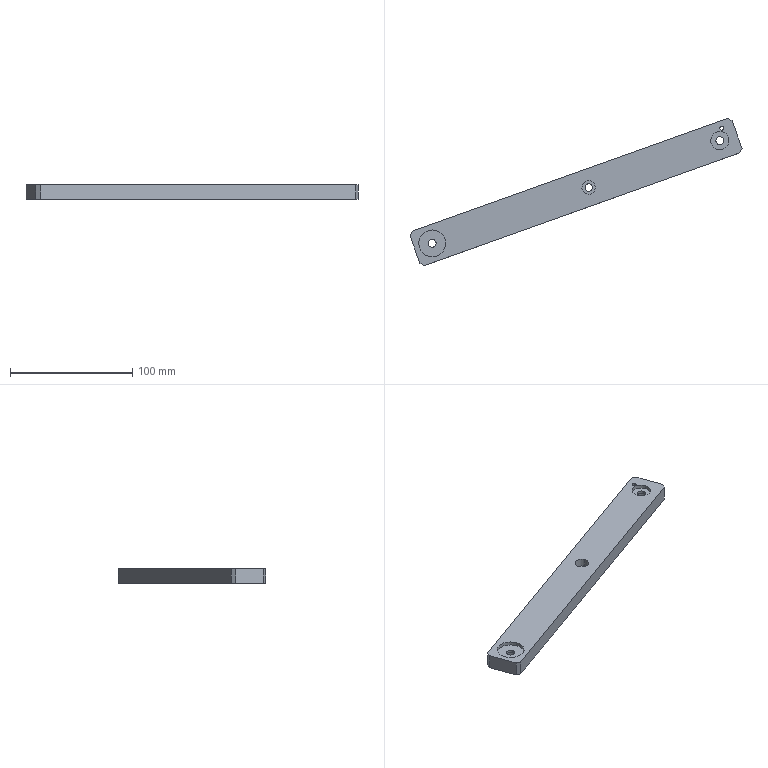Component | SolidWorks | JYTBJ-HeaderBrakeLever-1 | 1 solid | 36 faces | box 271.74 x 120.46 x 12 mm | volume 96229 mm3 | cylinder 20 | plane 16 | commonest cylinder face diameters 11 x6 6.6 x4 3.3 x2 16 x2 22 x2 15 x2 6 x2
build123d program:
from build123d import *

# Parameters (mm, degrees)
SKETCH1_W                                            = 280
SKETCH1_H                                            = 30
BOSS_EXTRUDE1_DEPTH                                  = 12
HOLE_SIZE_ACCORDING_TO_THE_TYPE_OF_HEXAG_D           = 6.6
HOLE_SIZE_ACCORDING_TO_THE_TYPE_OF_HEXAG_CBORE_D     = 11
HOLE_SIZE_ACCORDING_TO_THE_TYPE_OF_HEXAG_CBORE_DEPTH = 6.8
HOLE_SIZE_ACCORDING_TO_THE_TYPE_OF_H_2_D             = 6
HOLE_SIZE_ACCORDING_TO_THE_TYPE_OF_H_2_CBORE_D       = 11
HOLE_SIZE_ACCORDING_TO_THE_TYPE_OF_H_2_CBORE_DEPTH   = 6.8
SKETCH8_R                                            = 7.5
SKETCH8_R_2                                          = 11
CUT_EXTRUDE1_DEPTH                                   = 3
SKETCH9_R                                            = 8
CUT_EXTRUDE2_DEPTH                                   = 2
M4_TAPPED_HOLE1_D                                    = 3.3
CHAMFER1_SIZE                                        = 3


with BuildPart() as part:
    # Sketch1 → Boss-Extrude1 (new body)
    with BuildSketch(Plane.XY):
        Rectangle(SKETCH1_W, SKETCH1_H)
    extrude(amount=BOSS_EXTRUDE1_DEPTH)

    # Hole Size according to the type of hexag (through all)
    with Locations(Plane(origin=(0, 0, 0), x_dir=(-1, 0, 0), z_dir=(0, 0, -1))):
        with Locations((-125, 0), (125, 0)):
            CounterBoreHole(HOLE_SIZE_ACCORDING_TO_THE_TYPE_OF_HEXAG_D / 2, HOLE_SIZE_ACCORDING_TO_THE_TYPE_OF_HEXAG_CBORE_D / 2, HOLE_SIZE_ACCORDING_TO_THE_TYPE_OF_HEXAG_CBORE_DEPTH)

    # Hole Size according to the type of h 2 (through all)
    with Locations(Plane.XY.offset(12)):
        with Locations((-11, 0)):
            CounterBoreHole(HOLE_SIZE_ACCORDING_TO_THE_TYPE_OF_H_2_D / 2, HOLE_SIZE_ACCORDING_TO_THE_TYPE_OF_H_2_CBORE_D / 2, HOLE_SIZE_ACCORDING_TO_THE_TYPE_OF_H_2_CBORE_DEPTH)

    # Sketch8 → Cut-Extrude1 (cut)
    with BuildSketch(Plane.XY.offset(12)):
        with Locations((-125, 0)):
            Circle(SKETCH8_R)
        with Locations((125, 0)):
            Circle(SKETCH8_R_2)
    extrude(amount=-CUT_EXTRUDE1_DEPTH, mode=Mode.SUBTRACT)

    # Sketch9 → Cut-Extrude2 (cut)
    with BuildSketch(Plane(origin=(0, 0, 0), x_dir=(-1, 0, 0), z_dir=(0, 0, -1))):
        with Locations((11, 0)):
            Circle(SKETCH9_R)
    extrude(amount=-CUT_EXTRUDE2_DEPTH, mode=Mode.SUBTRACT)

    # M4 Tapped Hole1 (through all)
    with Locations(Plane(origin=(0, 0, 0), x_dir=(-1, 0, 0), z_dir=(0, 0, -1))):
        with Locations((130, -9)):
            Hole(M4_TAPPED_HOLE1_D / 2)

    # Chamfer1
    chamfer1_edges = [part.edges().sort_by_distance(p)[0] for p in [
        (140, 15, 6),
        (140, -15, 6),
        (-140, -15, 6),
        (-140, 15, 6),
    ]]
    chamfer(chamfer1_edges, length=CHAMFER1_SIZE)


solid = part.part

# Placed as in the assembly
solid = solid.moved(Location((-81.985, 223.08, 9), (0, 0, -160.334)))
STEP:
#1=COLOUR_RGB('',0.7922,0.8196,0.9333);
#2=FILL_AREA_STYLE_COLOUR('',#1);
#3=FILL_AREA_STYLE('',(#2));
#4=SURFACE_STYLE_FILL_AREA(#3);
#5=SURFACE_SIDE_STYLE('',(#4));
#6=SURFACE_STYLE_USAGE(.BOTH.,#5);
#7=PRESENTATION_STYLE_ASSIGNMENT((#6));
#8=CARTESIAN_POINT('',(1.411,10.817,0.8268));
#9=VERTEX_POINT('',#8);
#10=CARTESIAN_POINT('',(1.534,10.861,0.8268));
#11=VERTEX_POINT('',#10);
#12=CARTESIAN_POINT('',(1.473,10.839,0.8268));
#13=DIRECTION('',(-0.,0.,-1.));
#14=DIRECTION('',(0.9417,0.3365,0.));
#15=AXIS2_PLACEMENT_3D('',#12,#13,#14);
#16=CIRCLE('',#15,0.06496);
#17=EDGE_CURVE('',#9,#11,#16,.T.);
#18=ORIENTED_EDGE('',*,*,#17,.F.);
#19=CARTESIAN_POINT('',(1.411,10.817,0.3543));
#20=VERTEX_POINT('',#19);
#21=CARTESIAN_POINT('',(1.411,10.817,0.3543));
#22=DIRECTION('',(-0.,0.,-1.));
#23=VECTOR('',#22,39.37);
#24=LINE('',#21,#23);
#25=EDGE_CURVE('',#9,#20,#24,.T.);
#26=ORIENTED_EDGE('',*,*,#25,.T.);
#27=CARTESIAN_POINT('',(1.534,10.861,0.3543));
#28=VERTEX_POINT('',#27);
#29=CARTESIAN_POINT('',(1.473,10.839,0.3543));
#30=DIRECTION('',(-0.,0.,-1.));
#31=DIRECTION('',(0.9417,0.3365,0.));
#32=AXIS2_PLACEMENT_3D('',#29,#30,#31);
#33=CIRCLE('',#32,0.06496);
#34=EDGE_CURVE('',#20,#28,#33,.T.);
#35=ORIENTED_EDGE('',*,*,#34,.T.);
#36=CARTESIAN_POINT('',(1.534,10.861,0.3543));
#37=DIRECTION('',(-0.,0.,-1.));
#38=VECTOR('',#37,39.37);
#39=LINE('',#36,#38);
#40=EDGE_CURVE('',#11,#28,#39,.T.);
#41=ORIENTED_EDGE('',*,*,#40,.F.);
#42=EDGE_LOOP('',(#18,#26,#35,#41));
#43=FACE_OUTER_BOUND('',#42,.T.);
#44=CARTESIAN_POINT('',(1.473,10.839,0.3543));
#45=DIRECTION('',(-0.,0.,-1.));
#46=DIRECTION('',(0.9417,0.3365,0.));
#47=AXIS2_PLACEMENT_3D('',#44,#45,#46);
#48=CYLINDRICAL_SURFACE('',#47,0.06496);
#49=ADVANCED_FACE('',(#43),#48,.F.);
#50=CARTESIAN_POINT('',(-3.117,8.822,0.4331));
#51=VERTEX_POINT('',#50);
#52=CARTESIAN_POINT('',(-2.523,9.034,0.4331));
#53=VERTEX_POINT('',#52);
#54=CARTESIAN_POINT('',(-2.82,8.928,0.4331));
#55=DIRECTION('',(-0.,0.,-1.));
#56=DIRECTION('',(0.9417,0.3365,0.));
#57=AXIS2_PLACEMENT_3D('',#54,#55,#56);
#58=CIRCLE('',#57,0.315);
#59=EDGE_CURVE('',#51,#53,#58,.T.);
#60=ORIENTED_EDGE('',*,*,#59,.F.);
#61=CARTESIAN_POINT('',(-3.117,8.822,0.3543));
#62=VERTEX_POINT('',#61);
#63=CARTESIAN_POINT('',(-3.117,8.822,0.4331));
#64=DIRECTION('',(-0.,0.,-1.));
#65=VECTOR('',#64,39.37);
#66=LINE('',#63,#65);
#67=EDGE_CURVE('',#51,#62,#66,.T.);
#68=ORIENTED_EDGE('',*,*,#67,.T.);
#69=CARTESIAN_POINT('',(-2.523,9.034,0.3543));
#70=VERTEX_POINT('',#69);
#71=CARTESIAN_POINT('',(-2.82,8.928,0.3543));
#72=DIRECTION('',(-0.,0.,-1.));
#73=DIRECTION('',(0.9417,0.3365,0.));
#74=AXIS2_PLACEMENT_3D('',#71,#72,#73);
#75=CIRCLE('',#74,0.315);
#76=EDGE_CURVE('',#62,#70,#75,.T.);
#77=ORIENTED_EDGE('',*,*,#76,.T.);
#78=CARTESIAN_POINT('',(-2.523,9.034,0.4331));
#79=DIRECTION('',(-0.,0.,-1.));
#80=VECTOR('',#79,39.37);
#81=LINE('',#78,#80);
#82=EDGE_CURVE('',#53,#70,#81,.T.);
#83=ORIENTED_EDGE('',*,*,#82,.F.);
#84=EDGE_LOOP('',(#60,#68,#77,#83));
#85=FACE_OUTER_BOUND('',#84,.T.);
#86=CARTESIAN_POINT('',(-2.82,8.928,0.4331));
#87=DIRECTION('',(-0.,0.,-1.));
#88=DIRECTION('',(0.9417,0.3365,0.));
#89=AXIS2_PLACEMENT_3D('',#86,#87,#88);
#90=CYLINDRICAL_SURFACE('',#89,0.315);
#91=ADVANCED_FACE('',(#85),#90,.F.);
#92=CARTESIAN_POINT('',(-7.454,7.272,0.7087));
#93=VERTEX_POINT('',#92);
#94=CARTESIAN_POINT('',(-8.27,6.981,0.7087));
#95=VERTEX_POINT('',#94);
#96=CARTESIAN_POINT('',(-7.862,7.126,0.7087));
#97=DIRECTION('',(0.,-0.,1.));
#98=DIRECTION('',(-0.9417,-0.3365,0.));
#99=AXIS2_PLACEMENT_3D('',#96,#97,#98);
#100=CIRCLE('',#99,0.4331);
#101=EDGE_CURVE('',#93,#95,#100,.T.);
#102=ORIENTED_EDGE('',*,*,#101,.F.);
#103=CARTESIAN_POINT('',(-7.454,7.272,0.8268));
#104=VERTEX_POINT('',#103);
#105=CARTESIAN_POINT('',(-7.454,7.272,0.7087));
#106=DIRECTION('',(0.,-0.,1.));
#107=VECTOR('',#106,39.37);
#108=LINE('',#105,#107);
#109=EDGE_CURVE('',#93,#104,#108,.T.);
#110=ORIENTED_EDGE('',*,*,#109,.T.);
#111=CARTESIAN_POINT('',(-8.27,6.981,0.8268));
#112=VERTEX_POINT('',#111);
#113=CARTESIAN_POINT('',(-7.862,7.126,0.8268));
#114=DIRECTION('',(0.,-0.,1.));
#115=DIRECTION('',(-0.9417,-0.3365,0.));
#116=AXIS2_PLACEMENT_3D('',#113,#114,#115);
#117=CIRCLE('',#116,0.4331);
#118=EDGE_CURVE('',#104,#112,#117,.T.);
#119=ORIENTED_EDGE('',*,*,#118,.T.);
#120=CARTESIAN_POINT('',(-8.27,6.981,0.7087));
#121=DIRECTION('',(0.,-0.,1.));
#122=VECTOR('',#121,39.37);
#123=LINE('',#120,#122);
#124=EDGE_CURVE('',#95,#112,#123,.T.);
#125=ORIENTED_EDGE('',*,*,#124,.F.);
#126=EDGE_LOOP('',(#102,#110,#119,#125));
#127=FACE_OUTER_BOUND('',#126,.T.);
#128=CARTESIAN_POINT('',(-7.862,7.126,0.7087));
#129=DIRECTION('',(0.,-0.,1.));
#130=DIRECTION('',(-0.9417,-0.3365,0.));
#131=AXIS2_PLACEMENT_3D('',#128,#129,#130);
#132=CYLINDRICAL_SURFACE('',#131,0.4331);
#133=ADVANCED_FACE('',(#127),#132,.F.);
#134=CARTESIAN_POINT('',(1.685,10.538,0.7087));
#135=VERTEX_POINT('',#134);
#136=CARTESIAN_POINT('',(1.128,10.339,0.7087));
#137=VERTEX_POINT('',#136);
#138=CARTESIAN_POINT('',(1.406,10.439,0.7087));
#139=DIRECTION('',(0.,-0.,1.));
#140=DIRECTION('',(-0.9417,-0.3365,0.));
#141=AXIS2_PLACEMENT_3D('',#138,#139,#140);
#142=CIRCLE('',#141,0.2953);
#143=EDGE_CURVE('',#135,#137,#142,.T.);
#144=ORIENTED_EDGE('',*,*,#143,.F.);
#145=CARTESIAN_POINT('',(1.685,10.538,0.8268));
#146=VERTEX_POINT('',#145);
#147=CARTESIAN_POINT('',(1.685,10.538,0.7087));
#148=DIRECTION('',(0.,-0.,1.));
#149=VECTOR('',#148,39.37);
#150=LINE('',#147,#149);
#151=EDGE_CURVE('',#135,#146,#150,.T.);
#152=ORIENTED_EDGE('',*,*,#151,.T.);
#153=CARTESIAN_POINT('',(1.128,10.339,0.8268));
#154=VERTEX_POINT('',#153);
#155=CARTESIAN_POINT('',(1.406,10.439,0.8268));
#156=DIRECTION('',(0.,-0.,1.));
#157=DIRECTION('',(-0.9417,-0.3365,0.));
#158=AXIS2_PLACEMENT_3D('',#155,#156,#157);
#159=CIRCLE('',#158,0.2953);
#160=EDGE_CURVE('',#146,#154,#159,.T.);
#161=ORIENTED_EDGE('',*,*,#160,.T.);
#162=CARTESIAN_POINT('',(1.128,10.339,0.7087));
#163=DIRECTION('',(0.,-0.,1.));
#164=VECTOR('',#163,39.37);
#165=LINE('',#162,#164);
#166=EDGE_CURVE('',#137,#154,#165,.T.);
#167=ORIENTED_EDGE('',*,*,#166,.F.);
#168=EDGE_LOOP('',(#144,#152,#161,#167));
#169=FACE_OUTER_BOUND('',#168,.T.);
#170=CARTESIAN_POINT('',(1.406,10.439,0.7087));
#171=DIRECTION('',(0.,-0.,1.));
#172=DIRECTION('',(-0.9417,-0.3365,0.));
#173=AXIS2_PLACEMENT_3D('',#170,#171,#172);
#174=CYLINDRICAL_SURFACE('',#173,0.2953);
#175=ADVANCED_FACE('',(#169),#174,.F.);
#176=CARTESIAN_POINT('',(-2.616,9.001,0.5591));
#177=VERTEX_POINT('',#176);
#178=CARTESIAN_POINT('',(-3.024,8.856,0.5591));
#179=VERTEX_POINT('',#178);
#180=CARTESIAN_POINT('',(-2.82,8.928,0.5591));
#181=DIRECTION('',(0.,-0.,1.));
#182=DIRECTION('',(-0.9417,-0.3365,0.));
#183=AXIS2_PLACEMENT_3D('',#180,#181,#182);
#184=CIRCLE('',#183,0.2165);
#185=EDGE_CURVE('',#177,#179,#184,.T.);
#186=ORIENTED_EDGE('',*,*,#185,.F.);
#187=CARTESIAN_POINT('',(-2.616,9.001,0.8268));
#188=VERTEX_POINT('',#187);
#189=CARTESIAN_POINT('',(-2.616,9.001,0.8268));
#190=DIRECTION('',(0.,-0.,1.));
#191=VECTOR('',#190,39.37);
#192=LINE('',#189,#191);
#193=EDGE_CURVE('',#177,#188,#192,.T.);
#194=ORIENTED_EDGE('',*,*,#193,.T.);
#195=CARTESIAN_POINT('',(-3.024,8.856,0.8268));
#196=VERTEX_POINT('',#195);
#197=CARTESIAN_POINT('',(-2.82,8.928,0.8268));
#198=DIRECTION('',(0.,-0.,1.));
#199=DIRECTION('',(-0.9417,-0.3365,0.));
#200=AXIS2_PLACEMENT_3D('',#197,#198,#199);
#201=CIRCLE('',#200,0.2165);
#202=EDGE_CURVE('',#188,#196,#201,.T.);
#203=ORIENTED_EDGE('',*,*,#202,.T.);
#204=CARTESIAN_POINT('',(-3.024,8.856,0.8268));
#205=DIRECTION('',(0.,-0.,1.));
#206=VECTOR('',#205,39.37);
#207=LINE('',#204,#206);
#208=EDGE_CURVE('',#179,#196,#207,.T.);
#209=ORIENTED_EDGE('',*,*,#208,.F.);
#210=EDGE_LOOP('',(#186,#194,#203,#209));
#211=FACE_OUTER_BOUND('',#210,.T.);
#212=CARTESIAN_POINT('',(-2.82,8.928,0.8268));
#213=DIRECTION('',(0.,-0.,1.));
#214=DIRECTION('',(-0.9417,-0.3365,0.));
#215=AXIS2_PLACEMENT_3D('',#212,#213,#214);
#216=CYLINDRICAL_SURFACE('',#215,0.2165);
#217=ADVANCED_FACE('',(#211),#216,.F.);
#218=CARTESIAN_POINT('',(-8.066,7.054,0.622));
#219=VERTEX_POINT('',#218);
#220=CARTESIAN_POINT('',(-7.658,7.199,0.622));
#221=VERTEX_POINT('',#220);
#222=CARTESIAN_POINT('',(-7.862,7.126,0.622));
#223=DIRECTION('',(-0.,0.,-1.));
#224=DIRECTION('',(0.9417,0.3365,0.));
#225=AXIS2_PLACEMENT_3D('',#222,#223,#224);
#226=CIRCLE('',#225,0.2165);
#227=EDGE_CURVE('',#219,#221,#226,.T.);
#228=ORIENTED_EDGE('',*,*,#227,.F.);
#229=CARTESIAN_POINT('',(-8.066,7.054,0.3543));
#230=VERTEX_POINT('',#229);
#231=CARTESIAN_POINT('',(-8.066,7.054,0.3543));
#232=DIRECTION('',(-0.,0.,-1.));
#233=VECTOR('',#232,39.37);
#234=LINE('',#231,#233);
#235=EDGE_CURVE('',#219,#230,#234,.T.);
#236=ORIENTED_EDGE('',*,*,#235,.T.);
#237=CARTESIAN_POINT('',(-7.658,7.199,0.3543));
#238=VERTEX_POINT('',#237);
#239=CARTESIAN_POINT('',(-7.862,7.126,0.3543));
#240=DIRECTION('',(-0.,0.,-1.));
#241=DIRECTION('',(0.9417,0.3365,0.));
#242=AXIS2_PLACEMENT_3D('',#239,#240,#241);
#243=CIRCLE('',#242,0.2165);
#244=EDGE_CURVE('',#230,#238,#243,.T.);
#245=ORIENTED_EDGE('',*,*,#244,.T.);
#246=CARTESIAN_POINT('',(-7.658,7.199,0.3543));
#247=DIRECTION('',(-0.,0.,-1.));
#248=VECTOR('',#247,39.37);
#249=LINE('',#246,#248);
#250=EDGE_CURVE('',#221,#238,#249,.T.);
#251=ORIENTED_EDGE('',*,*,#250,.F.);
#252=EDGE_LOOP('',(#228,#236,#245,#251));
#253=FACE_OUTER_BOUND('',#252,.T.);
#254=CARTESIAN_POINT('',(-7.862,7.126,0.3543));
#255=DIRECTION('',(-0.,0.,-1.));
#256=DIRECTION('',(0.9417,0.3365,0.));
#257=AXIS2_PLACEMENT_3D('',#254,#255,#256);
#258=CYLINDRICAL_SURFACE('',#257,0.2165);
#259=ADVANCED_FACE('',(#253),#258,.F.);
#260=CARTESIAN_POINT('',(1.203,10.366,0.622));
#261=VERTEX_POINT('',#260);
#262=CARTESIAN_POINT('',(1.61,10.512,0.622));
#263=VERTEX_POINT('',#262);
#264=CARTESIAN_POINT('',(1.406,10.439,0.622));
#265=DIRECTION('',(-0.,0.,-1.));
#266=DIRECTION('',(0.9417,0.3365,0.));
#267=AXIS2_PLACEMENT_3D('',#264,#265,#266);
#268=CIRCLE('',#267,0.2165);
#269=EDGE_CURVE('',#261,#263,#268,.T.);
#270=ORIENTED_EDGE('',*,*,#269,.F.);
#271=CARTESIAN_POINT('',(1.203,10.366,0.3543));
#272=VERTEX_POINT('',#271);
#273=CARTESIAN_POINT('',(1.203,10.366,0.3543));
#274=DIRECTION('',(-0.,0.,-1.));
#275=VECTOR('',#274,39.37);
#276=LINE('',#273,#275);
#277=EDGE_CURVE('',#261,#272,#276,.T.);
#278=ORIENTED_EDGE('',*,*,#277,.T.);
#279=CARTESIAN_POINT('',(1.61,10.512,0.3543));
#280=VERTEX_POINT('',#279);
#281=CARTESIAN_POINT('',(1.406,10.439,0.3543));
#282=DIRECTION('',(-0.,0.,-1.));
#283=DIRECTION('',(0.9417,0.3365,0.));
#284=AXIS2_PLACEMENT_3D('',#281,#282,#283);
#285=CIRCLE('',#284,0.2165);
#286=EDGE_CURVE('',#272,#280,#285,.T.);
#287=ORIENTED_EDGE('',*,*,#286,.T.);
#288=CARTESIAN_POINT('',(1.61,10.512,0.3543));
#289=DIRECTION('',(-0.,0.,-1.));
#290=VECTOR('',#289,39.37);
#291=LINE('',#288,#290);
#292=EDGE_CURVE('',#263,#280,#291,.T.);
#293=ORIENTED_EDGE('',*,*,#292,.F.);
#294=EDGE_LOOP('',(#270,#278,#287,#293));
#295=FACE_OUTER_BOUND('',#294,.T.);
#296=CARTESIAN_POINT('',(1.406,10.439,0.3543));
#297=DIRECTION('',(-0.,0.,-1.));
#298=DIRECTION('',(0.9417,0.3365,0.));
#299=AXIS2_PLACEMENT_3D('',#296,#297,#298);
#300=CYLINDRICAL_SURFACE('',#299,0.2165);
#301=ADVANCED_FACE('',(#295),#300,.F.);
#302=CARTESIAN_POINT('',(1.284,10.395,0.7087));
#303=VERTEX_POINT('',#302);
#304=CARTESIAN_POINT('',(1.529,10.483,0.7087));
#305=VERTEX_POINT('',#304);
#306=CARTESIAN_POINT('',(1.406,10.439,0.7087));
#307=DIRECTION('',(-0.,0.,-1.));
#308=DIRECTION('',(-0.9417,-0.3365,0.));
#309=AXIS2_PLACEMENT_3D('',#306,#307,#308);
#310=CIRCLE('',#309,0.1299);
#311=EDGE_CURVE('',#303,#305,#310,.T.);
#312=ORIENTED_EDGE('',*,*,#311,.F.);
#313=CARTESIAN_POINT('',(1.284,10.395,0.622));
#314=VERTEX_POINT('',#313);
#315=CARTESIAN_POINT('',(1.284,10.395,0.3543));
#316=DIRECTION('',(-0.,0.,-1.));
#317=VECTOR('',#316,39.37);
#318=LINE('',#315,#317);
#319=EDGE_CURVE('',#303,#314,#318,.T.);
#320=ORIENTED_EDGE('',*,*,#319,.T.);
#321=CARTESIAN_POINT('',(1.529,10.483,0.622));
#322=VERTEX_POINT('',#321);
#323=CARTESIAN_POINT('',(1.406,10.439,0.622));
#324=DIRECTION('',(-0.,0.,-1.));
#325=DIRECTION('',(0.9417,0.3365,0.));
#326=AXIS2_PLACEMENT_3D('',#323,#324,#325);
#327=CIRCLE('',#326,0.1299);
#328=EDGE_CURVE('',#314,#322,#327,.T.);
#329=ORIENTED_EDGE('',*,*,#328,.T.);
#330=CARTESIAN_POINT('',(1.529,10.483,0.3543));
#331=DIRECTION('',(-0.,0.,-1.));
#332=VECTOR('',#331,39.37);
#333=LINE('',#330,#332);
#334=EDGE_CURVE('',#305,#322,#333,.T.);
#335=ORIENTED_EDGE('',*,*,#334,.F.);
#336=EDGE_LOOP('',(#312,#320,#329,#335));
#337=FACE_OUTER_BOUND('',#336,.T.);
#338=CARTESIAN_POINT('',(1.406,10.439,0.3543));
#339=DIRECTION('',(-0.,0.,-1.));
#340=DIRECTION('',(0.9417,0.3365,0.));
#341=AXIS2_PLACEMENT_3D('',#338,#339,#340);
#342=CYLINDRICAL_SURFACE('',#341,0.1299);
#343=ADVANCED_FACE('',(#337),#342,.F.);
#344=CARTESIAN_POINT('',(-7.984,7.083,0.7087));
#345=VERTEX_POINT('',#344);
#346=CARTESIAN_POINT('',(-7.74,7.17,0.7087));
#347=VERTEX_POINT('',#346);
#348=CARTESIAN_POINT('',(-7.862,7.126,0.7087));
#349=DIRECTION('',(-0.,0.,-1.));
#350=DIRECTION('',(-0.9417,-0.3365,0.));
#351=AXIS2_PLACEMENT_3D('',#348,#349,#350);
#352=CIRCLE('',#351,0.1299);
#353=EDGE_CURVE('',#345,#347,#352,.T.);
#354=ORIENTED_EDGE('',*,*,#353,.F.);
#355=CARTESIAN_POINT('',(-7.984,7.083,0.622));
#356=VERTEX_POINT('',#355);
#357=CARTESIAN_POINT('',(-7.984,7.083,0.3543));
#358=DIRECTION('',(-0.,0.,-1.));
#359=VECTOR('',#358,39.37);
#360=LINE('',#357,#359);
#361=EDGE_CURVE('',#345,#356,#360,.T.);
#362=ORIENTED_EDGE('',*,*,#361,.T.);
#363=CARTESIAN_POINT('',(-7.74,7.17,0.622));
#364=VERTEX_POINT('',#363);
#365=CARTESIAN_POINT('',(-7.862,7.126,0.622));
#366=DIRECTION('',(-0.,0.,-1.));
#367=DIRECTION('',(0.9417,0.3365,0.));
#368=AXIS2_PLACEMENT_3D('',#365,#366,#367);
#369=CIRCLE('',#368,0.1299);
#370=EDGE_CURVE('',#356,#364,#369,.T.);
#371=ORIENTED_EDGE('',*,*,#370,.T.);
#372=CARTESIAN_POINT('',(-7.74,7.17,0.3543));
#373=DIRECTION('',(-0.,0.,-1.));
#374=VECTOR('',#373,39.37);
#375=LINE('',#372,#374);
#376=EDGE_CURVE('',#347,#364,#375,.T.);
#377=ORIENTED_EDGE('',*,*,#376,.F.);
#378=EDGE_LOOP('',(#354,#362,#371,#377));
#379=FACE_OUTER_BOUND('',#378,.T.);
#380=CARTESIAN_POINT('',(-7.862,7.126,0.3543));
#381=DIRECTION('',(-0.,0.,-1.));
#382=DIRECTION('',(0.9417,0.3365,0.));
#383=AXIS2_PLACEMENT_3D('',#380,#381,#382);
#384=CYLINDRICAL_SURFACE('',#383,0.1299);
#385=ADVANCED_FACE('',(#379),#384,.F.);
#386=CARTESIAN_POINT('',(-2.709,8.968,0.4331));
#387=VERTEX_POINT('',#386);
#388=CARTESIAN_POINT('',(-2.931,8.889,0.4331));
#389=VERTEX_POINT('',#388);
#390=CARTESIAN_POINT('',(-2.82,8.928,0.4331));
#391=DIRECTION('',(0.,-0.,1.));
#392=DIRECTION('',(0.9417,0.3365,0.));
#393=AXIS2_PLACEMENT_3D('',#390,#391,#392);
#394=CIRCLE('',#393,0.1181);
#395=EDGE_CURVE('',#387,#389,#394,.T.);
#396=ORIENTED_EDGE('',*,*,#395,.F.);
#397=CARTESIAN_POINT('',(-2.709,8.968,0.5591));
#398=VERTEX_POINT('',#397);
#399=CARTESIAN_POINT('',(-2.709,8.968,0.8268));
#400=DIRECTION('',(0.,-0.,1.));
#401=VECTOR('',#400,39.37);
#402=LINE('',#399,#401);
#403=EDGE_CURVE('',#387,#398,#402,.T.);
#404=ORIENTED_EDGE('',*,*,#403,.T.);
#405=CARTESIAN_POINT('',(-2.931,8.889,0.5591));
#406=VERTEX_POINT('',#405);
#407=CARTESIAN_POINT('',(-2.82,8.928,0.5591));
#408=DIRECTION('',(0.,-0.,1.));
#409=DIRECTION('',(-0.9417,-0.3365,0.));
#410=AXIS2_PLACEMENT_3D('',#407,#408,#409);
#411=CIRCLE('',#410,0.1181);
#412=EDGE_CURVE('',#398,#406,#411,.T.);
#413=ORIENTED_EDGE('',*,*,#412,.T.);
#414=CARTESIAN_POINT('',(-2.931,8.889,0.8268));
#415=DIRECTION('',(0.,-0.,1.));
#416=VECTOR('',#415,39.37);
#417=LINE('',#414,#416);
#418=EDGE_CURVE('',#389,#406,#417,.T.);
#419=ORIENTED_EDGE('',*,*,#418,.F.);
#420=EDGE_LOOP('',(#396,#404,#413,#419));
#421=FACE_OUTER_BOUND('',#420,.T.);
#422=CARTESIAN_POINT('',(-2.82,8.928,0.8268));
#423=DIRECTION('',(0.,-0.,1.));
#424=DIRECTION('',(-0.9417,-0.3365,0.));
#425=AXIS2_PLACEMENT_3D('',#422,#423,#424);
#426=CYLINDRICAL_SURFACE('',#425,0.1181);
#427=ADVANCED_FACE('',(#421),#426,.F.);
#428=ORIENTED_EDGE('',*,*,#403,.F.);
#429=CARTESIAN_POINT('',(-2.82,8.928,0.4331));
#430=DIRECTION('',(0.,-0.,1.));
#431=DIRECTION('',(0.9417,0.3365,0.));
#432=AXIS2_PLACEMENT_3D('',#429,#430,#431);
#433=CIRCLE('',#432,0.1181);
#434=EDGE_CURVE('',#389,#387,#433,.T.);
#435=ORIENTED_EDGE('',*,*,#434,.F.);
#436=ORIENTED_EDGE('',*,*,#418,.T.);
#437=CARTESIAN_POINT('',(-2.82,8.928,0.5591));
#438=DIRECTION('',(0.,-0.,1.));
#439=DIRECTION('',(-0.9417,-0.3365,0.));
#440=AXIS2_PLACEMENT_3D('',#437,#438,#439);
#441=CIRCLE('',#440,0.1181);
#442=EDGE_CURVE('',#406,#398,#441,.T.);
#443=ORIENTED_EDGE('',*,*,#442,.T.);
#444=EDGE_LOOP('',(#428,#435,#436,#443));
#445=FACE_OUTER_BOUND('',#444,.T.);
#446=CARTESIAN_POINT('',(-2.82,8.928,0.8268));
#447=DIRECTION('',(0.,-0.,1.));
#448=DIRECTION('',(-0.9417,-0.3365,0.));
#449=AXIS2_PLACEMENT_3D('',#446,#447,#448);
#450=CYLINDRICAL_SURFACE('',#449,0.1181);
#451=ADVANCED_FACE('',(#445),#450,.F.);
#452=ORIENTED_EDGE('',*,*,#361,.F.);
#453=CARTESIAN_POINT('',(-7.862,7.126,0.7087));
#454=DIRECTION('',(-0.,0.,-1.));
#455=DIRECTION('',(-0.9417,-0.3365,0.));
#456=AXIS2_PLACEMENT_3D('',#453,#454,#455);
#457=CIRCLE('',#456,0.1299);
#458=EDGE_CURVE('',#347,#345,#457,.T.);
#459=ORIENTED_EDGE('',*,*,#458,.F.);
#460=ORIENTED_EDGE('',*,*,#376,.T.);
#461=CARTESIAN_POINT('',(-7.862,7.126,0.622));
#462=DIRECTION('',(-0.,0.,-1.));
#463=DIRECTION('',(0.9417,0.3365,0.));
#464=AXIS2_PLACEMENT_3D('',#461,#462,#463);
#465=CIRCLE('',#464,0.1299);
#466=EDGE_CURVE('',#364,#356,#465,.T.);
#467=ORIENTED_EDGE('',*,*,#466,.T.);
#468=EDGE_LOOP('',(#452,#459,#460,#467));
#469=FACE_OUTER_BOUND('',#468,.T.);
#470=CARTESIAN_POINT('',(-7.862,7.126,0.3543));
#471=DIRECTION('',(-0.,0.,-1.));
#472=DIRECTION('',(0.9417,0.3365,0.));
#473=AXIS2_PLACEMENT_3D('',#470,#471,#472);
#474=CYLINDRICAL_SURFACE('',#473,0.1299);
#475=ADVANCED_FACE('',(#469),#474,.F.);
#476=ORIENTED_EDGE('',*,*,#319,.F.);
#477=CARTESIAN_POINT('',(1.406,10.439,0.7087));
#478=DIRECTION('',(-0.,0.,-1.));
#479=DIRECTION('',(-0.9417,-0.3365,0.));
#480=AXIS2_PLACEMENT_3D('',#477,#478,#479);
#481=CIRCLE('',#480,0.1299);
#482=EDGE_CURVE('',#305,#303,#481,.T.);
#483=ORIENTED_EDGE('',*,*,#482,.F.);
#484=ORIENTED_EDGE('',*,*,#334,.T.);
#485=CARTESIAN_POINT('',(1.406,10.439,0.622));
#486=DIRECTION('',(-0.,0.,-1.));
#487=DIRECTION('',(0.9417,0.3365,0.));
#488=AXIS2_PLACEMENT_3D('',#485,#486,#487);
#489=CIRCLE('',#488,0.1299);
#490=EDGE_CURVE('',#322,#314,#489,.T.);
#491=ORIENTED_EDGE('',*,*,#490,.T.);
#492=EDGE_LOOP('',(#476,#483,#484,#491));
#493=FACE_OUTER_BOUND('',#492,.T.);
#494=CARTESIAN_POINT('',(1.406,10.439,0.3543));
#495=DIRECTION('',(-0.,0.,-1.));
#496=DIRECTION('',(0.9417,0.3365,0.));
#497=AXIS2_PLACEMENT_3D('',#494,#495,#496);
#498=CYLINDRICAL_SURFACE('',#497,0.1299);
#499=ADVANCED_FACE('',(#493),#498,.F.);
#500=CARTESIAN_POINT('',(-8.108,6.411,0.8268));
#501=VERTEX_POINT('',#500);
#502=CARTESIAN_POINT('',(2.05,10.042,0.8268));
#503=VERTEX_POINT('',#502);
#504=CARTESIAN_POINT('',(2.161,10.081,0.8268));
#505=DIRECTION('',(0.9417,0.3365,-0.));
#506=VECTOR('',#505,39.37);
#507=LINE('',#504,#506);
#508=EDGE_CURVE('',#501,#503,#507,.T.);
#509=ORIENTED_EDGE('',*,*,#508,.F.);
#510=CARTESIAN_POINT('',(-8.108,6.411,0.3543));
#511=VERTEX_POINT('',#510);
#512=CARTESIAN_POINT('',(-8.108,6.411,0.8268));
#513=DIRECTION('',(-0.,0.,-1.));
#514=VECTOR('',#513,39.37);
#515=LINE('',#512,#514);
#516=EDGE_CURVE('',#501,#511,#515,.T.);
#517=ORIENTED_EDGE('',*,*,#516,.T.);
#518=CARTESIAN_POINT('',(2.05,10.042,0.3543));
#519=VERTEX_POINT('',#518);
#520=CARTESIAN_POINT('',(2.161,10.081,0.3543));
#521=DIRECTION('',(0.9417,0.3365,-0.));
#522=VECTOR('',#521,39.37);
#523=LINE('',#520,#522);
#524=EDGE_CURVE('',#511,#519,#523,.T.);
#525=ORIENTED_EDGE('',*,*,#524,.T.);
#526=CARTESIAN_POINT('',(2.05,10.042,0.8268));
#527=DIRECTION('',(0.,-0.,1.));
#528=VECTOR('',#527,39.37);
#529=LINE('',#526,#528);
#530=EDGE_CURVE('',#519,#503,#529,.T.);
#531=ORIENTED_EDGE('',*,*,#530,.T.);
#532=EDGE_LOOP('',(#509,#517,#525,#531));
#533=FACE_OUTER_BOUND('',#532,.T.);
#534=CARTESIAN_POINT('',(2.161,10.081,0.8268));
#535=DIRECTION('',(-0.3365,0.9417,0.));
#536=DIRECTION('',(-0.,0.,-1.));
#537=AXIS2_PLACEMENT_3D('',#534,#535,#536);
#538=PLANE('',#537);
#539=ADVANCED_FACE('',(#533),#538,.F.);
#540=CARTESIAN_POINT('',(2.122,10.193,0.3543));
#541=VERTEX_POINT('',#540);
#542=CARTESIAN_POINT('',(1.804,11.082,0.3543));
#543=VERTEX_POINT('',#542);
#544=CARTESIAN_POINT('',(2.161,10.081,0.3543));
#545=DIRECTION('',(-0.3365,0.9417,0.));
#546=VECTOR('',#545,39.37);
#547=LINE('',#544,#546);
#548=EDGE_CURVE('',#541,#543,#547,.T.);
#549=ORIENTED_EDGE('',*,*,#548,.T.);
#550=CARTESIAN_POINT('',(1.804,11.082,0.8268));
#551=VERTEX_POINT('',#550);
#552=CARTESIAN_POINT('',(1.804,11.082,0.8268));
#553=DIRECTION('',(0.,-0.,1.));
#554=VECTOR('',#553,39.37);
#555=LINE('',#552,#554);
#556=EDGE_CURVE('',#543,#551,#555,.T.);
#557=ORIENTED_EDGE('',*,*,#556,.T.);
#558=CARTESIAN_POINT('',(2.122,10.193,0.8268));
#559=VERTEX_POINT('',#558);
#560=CARTESIAN_POINT('',(2.161,10.081,0.8268));
#561=DIRECTION('',(-0.3365,0.9417,0.));
#562=VECTOR('',#561,39.37);
#563=LINE('',#560,#562);
#564=EDGE_CURVE('',#559,#551,#563,.T.);
#565=ORIENTED_EDGE('',*,*,#564,.F.);
#566=CARTESIAN_POINT('',(2.122,10.193,0.8268));
#567=DIRECTION('',(-0.,0.,-1.));
#568=VECTOR('',#567,39.37);
#569=LINE('',#566,#568);
#570=EDGE_CURVE('',#559,#541,#569,.T.);
#571=ORIENTED_EDGE('',*,*,#570,.T.);
#572=EDGE_LOOP('',(#549,#557,#565,#571));
#573=FACE_OUTER_BOUND('',#572,.T.);
#574=CARTESIAN_POINT('',(2.161,10.081,0.8268));
#575=DIRECTION('',(-0.9417,-0.3365,0.));
#576=DIRECTION('',(-0.,0.,-1.));
#577=AXIS2_PLACEMENT_3D('',#574,#575,#576);
#578=PLANE('',#577);
#579=ADVANCED_FACE('',(#573),#578,.F.);
#580=CARTESIAN_POINT('',(1.653,11.154,0.3543));
#581=VERTEX_POINT('',#580);
#582=CARTESIAN_POINT('',(-8.506,7.524,0.3543));
#583=VERTEX_POINT('',#582);
#584=CARTESIAN_POINT('',(1.764,11.194,0.3543));
#585=DIRECTION('',(-0.9417,-0.3365,0.));
#586=VECTOR('',#585,39.37);
#587=LINE('',#584,#586);
#588=EDGE_CURVE('',#581,#583,#587,.T.);
#589=ORIENTED_EDGE('',*,*,#588,.T.);
#590=CARTESIAN_POINT('',(-8.506,7.524,0.8268));
#591=VERTEX_POINT('',#590);
#592=CARTESIAN_POINT('',(-8.506,7.524,0.8268));
#593=DIRECTION('',(0.,-0.,1.));
#594=VECTOR('',#593,39.37);
#595=LINE('',#592,#594);
#596=EDGE_CURVE('',#583,#591,#595,.T.);
#597=ORIENTED_EDGE('',*,*,#596,.T.);
#598=CARTESIAN_POINT('',(1.653,11.154,0.8268));
#599=VERTEX_POINT('',#598);
#600=CARTESIAN_POINT('',(1.764,11.194,0.8268));
#601=DIRECTION('',(-0.9417,-0.3365,0.));
#602=VECTOR('',#601,39.37);
#603=LINE('',#600,#602);
#604=EDGE_CURVE('',#599,#591,#603,.T.);
#605=ORIENTED_EDGE('',*,*,#604,.F.);
#606=CARTESIAN_POINT('',(1.653,11.154,0.8268));
#607=DIRECTION('',(-0.,0.,-1.));
#608=VECTOR('',#607,39.37);
#609=LINE('',#606,#608);
#610=EDGE_CURVE('',#599,#581,#609,.T.);
#611=ORIENTED_EDGE('',*,*,#610,.T.);
#612=EDGE_LOOP('',(#589,#597,#605,#611));
#613=FACE_OUTER_BOUND('',#612,.T.);
#614=CARTESIAN_POINT('',(1.764,11.194,0.8268));
#615=DIRECTION('',(0.3365,-0.9417,-0.));
#616=DIRECTION('',(0.,-0.,1.));
#617=AXIS2_PLACEMENT_3D('',#614,#615,#616);
#618=PLANE('',#617);
#619=ADVANCED_FACE('',(#613),#618,.F.);
#620=CARTESIAN_POINT('',(-8.577,7.373,0.8268));
#621=VERTEX_POINT('',#620);
#622=CARTESIAN_POINT('',(-8.259,6.483,0.8268));
#623=VERTEX_POINT('',#622);
#624=CARTESIAN_POINT('',(-8.219,6.372,0.8268));
#625=DIRECTION('',(0.3365,-0.9417,-0.));
#626=VECTOR('',#625,39.37);
#627=LINE('',#624,#626);
#628=EDGE_CURVE('',#621,#623,#627,.T.);
#629=ORIENTED_EDGE('',*,*,#628,.F.);
#630=CARTESIAN_POINT('',(-8.577,7.373,0.3543));
#631=VERTEX_POINT('',#630);
#632=CARTESIAN_POINT('',(-8.577,7.373,0.8268));
#633=DIRECTION('',(-0.,0.,-1.));
#634=VECTOR('',#633,39.37);
#635=LINE('',#632,#634);
#636=EDGE_CURVE('',#621,#631,#635,.T.);
#637=ORIENTED_EDGE('',*,*,#636,.T.);
#638=CARTESIAN_POINT('',(-8.259,6.483,0.3543));
#639=VERTEX_POINT('',#638);
#640=CARTESIAN_POINT('',(-8.219,6.372,0.3543));
#641=DIRECTION('',(0.3365,-0.9417,-0.));
#642=VECTOR('',#641,39.37);
#643=LINE('',#640,#642);
#644=EDGE_CURVE('',#631,#639,#643,.T.);
#645=ORIENTED_EDGE('',*,*,#644,.T.);
#646=CARTESIAN_POINT('',(-8.259,6.483,0.8268));
#647=DIRECTION('',(0.,-0.,1.));
#648=VECTOR('',#647,39.37);
#649=LINE('',#646,#648);
#650=EDGE_CURVE('',#639,#623,#649,.T.);
#651=ORIENTED_EDGE('',*,*,#650,.T.);
#652=EDGE_LOOP('',(#629,#637,#645,#651));
#653=FACE_OUTER_BOUND('',#652,.T.);
#654=CARTESIAN_POINT('',(-8.219,6.372,0.8268));
#655=DIRECTION('',(0.9417,0.3365,-0.));
#656=DIRECTION('',(0.,-0.,1.));
#657=AXIS2_PLACEMENT_3D('',#654,#655,#656);
#658=PLANE('',#657);
#659=ADVANCED_FACE('',(#653),#658,.F.);
#660=CARTESIAN_POINT('',(1.473,10.839,0.8268));
#661=DIRECTION('',(-0.,0.,-1.));
#662=DIRECTION('',(0.9417,0.3365,0.));
#663=AXIS2_PLACEMENT_3D('',#660,#661,#662);
#664=CIRCLE('',#663,0.06496);
#665=EDGE_CURVE('',#11,#9,#664,.T.);
#666=ORIENTED_EDGE('',*,*,#665,.T.);
#667=ORIENTED_EDGE('',*,*,#17,.T.);
#668=EDGE_LOOP('',(#666,#667));
#669=FACE_BOUND('',#668,.T.);
#670=CARTESIAN_POINT('',(-7.862,7.126,0.8268));
#671=DIRECTION('',(0.,-0.,1.));
#672=DIRECTION('',(-0.9417,-0.3365,0.));
#673=AXIS2_PLACEMENT_3D('',#670,#671,#672);
#674=CIRCLE('',#673,0.4331);
#675=EDGE_CURVE('',#112,#104,#674,.T.);
#676=ORIENTED_EDGE('',*,*,#675,.F.);
#677=ORIENTED_EDGE('',*,*,#118,.F.);
#678=EDGE_LOOP('',(#676,#677));
#679=FACE_BOUND('',#678,.T.);
#680=CARTESIAN_POINT('',(1.406,10.439,0.8268));
#681=DIRECTION('',(0.,-0.,1.));
#682=DIRECTION('',(-0.9417,-0.3365,0.));
#683=AXIS2_PLACEMENT_3D('',#680,#681,#682);
#684=CIRCLE('',#683,0.2953);
#685=EDGE_CURVE('',#154,#146,#684,.T.);
#686=ORIENTED_EDGE('',*,*,#685,.F.);
#687=ORIENTED_EDGE('',*,*,#160,.F.);
#688=EDGE_LOOP('',(#686,#687));
#689=FACE_BOUND('',#688,.T.);
#690=CARTESIAN_POINT('',(-2.82,8.928,0.8268));
#691=DIRECTION('',(0.,-0.,1.));
#692=DIRECTION('',(-0.9417,-0.3365,0.));
#693=AXIS2_PLACEMENT_3D('',#690,#691,#692);
#694=CIRCLE('',#693,0.2165);
#695=EDGE_CURVE('',#196,#188,#694,.T.);
#696=ORIENTED_EDGE('',*,*,#695,.F.);
#697=ORIENTED_EDGE('',*,*,#202,.F.);
#698=EDGE_LOOP('',(#696,#697));
#699=FACE_BOUND('',#698,.T.);
#700=ORIENTED_EDGE('',*,*,#604,.T.);
#701=CARTESIAN_POINT('',(-8.577,7.373,0.8268));
#702=DIRECTION('',(-0.4279,-0.9038,0.));
#703=VECTOR('',#702,39.37);
#704=LINE('',#701,#703);
#705=EDGE_CURVE('',#591,#621,#704,.T.);
#706=ORIENTED_EDGE('',*,*,#705,.T.);
#707=ORIENTED_EDGE('',*,*,#628,.T.);
#708=CARTESIAN_POINT('',(-8.108,6.411,0.8268));
#709=DIRECTION('',(0.9038,-0.4279,-0.));
#710=VECTOR('',#709,39.37);
#711=LINE('',#708,#710);
#712=EDGE_CURVE('',#623,#501,#711,.T.);
#713=ORIENTED_EDGE('',*,*,#712,.T.);
#714=ORIENTED_EDGE('',*,*,#508,.T.);
#715=CARTESIAN_POINT('',(2.122,10.193,0.8268));
#716=DIRECTION('',(0.4279,0.9038,-0.));
#717=VECTOR('',#716,39.37);
#718=LINE('',#715,#717);
#719=EDGE_CURVE('',#503,#559,#718,.T.);
#720=ORIENTED_EDGE('',*,*,#719,.T.);
#721=ORIENTED_EDGE('',*,*,#564,.T.);
#722=CARTESIAN_POINT('',(1.653,11.154,0.8268));
#723=DIRECTION('',(-0.9038,0.4279,0.));
#724=VECTOR('',#723,39.37);
#725=LINE('',#722,#724);
#726=EDGE_CURVE('',#551,#599,#725,.T.);
#727=ORIENTED_EDGE('',*,*,#726,.T.);
#728=EDGE_LOOP('',(#700,#706,#707,#713,#714,#720,#721,#727));
#729=FACE_OUTER_BOUND('',#728,.T.);
#730=CARTESIAN_POINT('',(-8.219,6.372,0.8268));
#731=DIRECTION('',(-0.,0.,-1.));
#732=DIRECTION('',(0.9417,0.3365,-0.));
#733=AXIS2_PLACEMENT_3D('',#730,#731,#732);
#734=PLANE('',#733);
#735=ADVANCED_FACE('',(#669,#679,#689,#699,#729),#734,.F.);
#736=CARTESIAN_POINT('',(1.473,10.839,0.3543));
#737=DIRECTION('',(-0.,0.,-1.));
#738=DIRECTION('',(0.9417,0.3365,0.));
#739=AXIS2_PLACEMENT_3D('',#736,#737,#738);
#740=CIRCLE('',#739,0.06496);
#741=EDGE_CURVE('',#28,#20,#740,.T.);
#742=ORIENTED_EDGE('',*,*,#741,.F.);
#743=ORIENTED_EDGE('',*,*,#34,.F.);
#744=EDGE_LOOP('',(#742,#743));
#745=FACE_BOUND('',#744,.T.);
#746=CARTESIAN_POINT('',(-2.82,8.928,0.3543));
#747=DIRECTION('',(-0.,0.,-1.));
#748=DIRECTION('',(0.9417,0.3365,0.));
#749=AXIS2_PLACEMENT_3D('',#746,#747,#748);
#750=CIRCLE('',#749,0.315);
#751=EDGE_CURVE('',#70,#62,#750,.T.);
#752=ORIENTED_EDGE('',*,*,#751,.F.);
#753=ORIENTED_EDGE('',*,*,#76,.F.);
#754=EDGE_LOOP('',(#752,#753));
#755=FACE_BOUND('',#754,.T.);
#756=CARTESIAN_POINT('',(-7.862,7.126,0.3543));
#757=DIRECTION('',(-0.,0.,-1.));
#758=DIRECTION('',(0.9417,0.3365,0.));
#759=AXIS2_PLACEMENT_3D('',#756,#757,#758);
#760=CIRCLE('',#759,0.2165);
#761=EDGE_CURVE('',#238,#230,#760,.T.);
#762=ORIENTED_EDGE('',*,*,#761,.F.);
#763=ORIENTED_EDGE('',*,*,#244,.F.);
#764=EDGE_LOOP('',(#762,#763));
#765=FACE_BOUND('',#764,.T.);
#766=CARTESIAN_POINT('',(1.406,10.439,0.3543));
#767=DIRECTION('',(-0.,0.,-1.));
#768=DIRECTION('',(0.9417,0.3365,0.));
#769=AXIS2_PLACEMENT_3D('',#766,#767,#768);
#770=CIRCLE('',#769,0.2165);
#771=EDGE_CURVE('',#280,#272,#770,.T.);
#772=ORIENTED_EDGE('',*,*,#771,.F.);
#773=ORIENTED_EDGE('',*,*,#286,.F.);
#774=EDGE_LOOP('',(#772,#773));
#775=FACE_BOUND('',#774,.T.);
#776=ORIENTED_EDGE('',*,*,#644,.F.);
#777=CARTESIAN_POINT('',(-8.899,6.693,0.3543));
#778=DIRECTION('',(0.4279,0.9038,-0.));
#779=VECTOR('',#778,39.37);
#780=LINE('',#777,#779);
#781=EDGE_CURVE('',#631,#583,#780,.T.);
#782=ORIENTED_EDGE('',*,*,#781,.T.);
#783=ORIENTED_EDGE('',*,*,#588,.F.);
#784=CARTESIAN_POINT('',(-4.562,14.096,0.3543));
#785=DIRECTION('',(0.9038,-0.4279,-0.));
#786=VECTOR('',#785,39.37);
#787=LINE('',#784,#786);
#788=EDGE_CURVE('',#581,#543,#787,.T.);
#789=ORIENTED_EDGE('',*,*,#788,.T.);
#790=ORIENTED_EDGE('',*,*,#548,.F.);
#791=CARTESIAN_POINT('',(-1.25,3.072,0.3543));
#792=DIRECTION('',(-0.4279,-0.9038,0.));
#793=VECTOR('',#792,39.37);
#794=LINE('',#791,#793);
#795=EDGE_CURVE('',#541,#519,#794,.T.);
#796=ORIENTED_EDGE('',*,*,#795,.T.);
#797=ORIENTED_EDGE('',*,*,#524,.F.);
#798=CARTESIAN_POINT('',(-8.184,6.447,0.3543));
#799=DIRECTION('',(-0.9038,0.4279,0.));
#800=VECTOR('',#799,39.37);
#801=LINE('',#798,#800);
#802=EDGE_CURVE('',#511,#639,#801,.T.);
#803=ORIENTED_EDGE('',*,*,#802,.T.);
#804=EDGE_LOOP('',(#776,#782,#783,#789,#790,#796,#797,#803));
#805=FACE_OUTER_BOUND('',#804,.T.);
#806=CARTESIAN_POINT('',(-8.219,6.372,0.3543));
#807=DIRECTION('',(-0.,0.,-1.));
#808=DIRECTION('',(0.9417,0.3365,-0.));
#809=AXIS2_PLACEMENT_3D('',#806,#807,#808);
#810=PLANE('',#809);
#811=ADVANCED_FACE('',(#745,#755,#765,#775,#805),#810,.T.);
#812=ORIENTED_EDGE('',*,*,#490,.F.);
#813=ORIENTED_EDGE('',*,*,#328,.F.);
#814=EDGE_LOOP('',(#812,#813));
#815=FACE_BOUND('',#814,.T.);
#816=CARTESIAN_POINT('',(1.406,10.439,0.622));
#817=DIRECTION('',(-0.,0.,-1.));
#818=DIRECTION('',(0.9417,0.3365,0.));
#819=AXIS2_PLACEMENT_3D('',#816,#817,#818);
#820=CIRCLE('',#819,0.2165);
#821=EDGE_CURVE('',#263,#261,#820,.T.);
#822=ORIENTED_EDGE('',*,*,#821,.T.);
#823=ORIENTED_EDGE('',*,*,#269,.T.);
#824=EDGE_LOOP('',(#822,#823));
#825=FACE_OUTER_BOUND('',#824,.T.);
#826=CARTESIAN_POINT('',(1.284,10.395,0.622));
#827=DIRECTION('',(0.,-0.,1.));
#828=DIRECTION('',(-0.9417,-0.3365,0.));
#829=AXIS2_PLACEMENT_3D('',#826,#827,#828);
#830=PLANE('',#829);
#831=ADVANCED_FACE('',(#815,#825),#830,.F.);
#832=ORIENTED_EDGE('',*,*,#277,.F.);
#833=ORIENTED_EDGE('',*,*,#821,.F.);
#834=ORIENTED_EDGE('',*,*,#292,.T.);
#835=ORIENTED_EDGE('',*,*,#771,.T.);
#836=EDGE_LOOP('',(#832,#833,#834,#835));
#837=FACE_OUTER_BOUND('',#836,.T.);
#838=CARTESIAN_POINT('',(1.406,10.439,0.3543));
#839=DIRECTION('',(-0.,0.,-1.));
#840=DIRECTION('',(0.9417,0.3365,0.));
#841=AXIS2_PLACEMENT_3D('',#838,#839,#840);
#842=CYLINDRICAL_SURFACE('',#841,0.2165);
#843=ADVANCED_FACE('',(#837),#842,.F.);
#844=ORIENTED_EDGE('',*,*,#466,.F.);
#845=ORIENTED_EDGE('',*,*,#370,.F.);
#846=EDGE_LOOP('',(#844,#845));
#847=FACE_BOUND('',#846,.T.);
#848=CARTESIAN_POINT('',(-7.862,7.126,0.622));
#849=DIRECTION('',(-0.,0.,-1.));
#850=DIRECTION('',(0.9417,0.3365,0.));
#851=AXIS2_PLACEMENT_3D('',#848,#849,#850);
#852=CIRCLE('',#851,0.2165);
#853=EDGE_CURVE('',#221,#219,#852,.T.);
#854=ORIENTED_EDGE('',*,*,#853,.T.);
#855=ORIENTED_EDGE('',*,*,#227,.T.);
#856=EDGE_LOOP('',(#854,#855));
#857=FACE_OUTER_BOUND('',#856,.T.);
#858=CARTESIAN_POINT('',(-7.984,7.083,0.622));
#859=DIRECTION('',(0.,-0.,1.));
#860=DIRECTION('',(-0.9417,-0.3365,0.));
#861=AXIS2_PLACEMENT_3D('',#858,#859,#860);
#862=PLANE('',#861);
#863=ADVANCED_FACE('',(#847,#857),#862,.F.);
#864=ORIENTED_EDGE('',*,*,#235,.F.);
#865=ORIENTED_EDGE('',*,*,#853,.F.);
#866=ORIENTED_EDGE('',*,*,#250,.T.);
#867=ORIENTED_EDGE('',*,*,#761,.T.);
#868=EDGE_LOOP('',(#864,#865,#866,#867));
#869=FACE_OUTER_BOUND('',#868,.T.);
#870=CARTESIAN_POINT('',(-7.862,7.126,0.3543));
#871=DIRECTION('',(-0.,0.,-1.));
#872=DIRECTION('',(0.9417,0.3365,0.));
#873=AXIS2_PLACEMENT_3D('',#870,#871,#872);
#874=CYLINDRICAL_SURFACE('',#873,0.2165);
#875=ADVANCED_FACE('',(#869),#874,.F.);
#876=ORIENTED_EDGE('',*,*,#442,.F.);
#877=ORIENTED_EDGE('',*,*,#412,.F.);
#878=EDGE_LOOP('',(#876,#877));
#879=FACE_BOUND('',#878,.T.);
#880=CARTESIAN_POINT('',(-2.82,8.928,0.5591));
#881=DIRECTION('',(0.,-0.,1.));
#882=DIRECTION('',(-0.9417,-0.3365,0.));
#883=AXIS2_PLACEMENT_3D('',#880,#881,#882);
#884=CIRCLE('',#883,0.2165);
#885=EDGE_CURVE('',#179,#177,#884,.T.);
#886=ORIENTED_EDGE('',*,*,#885,.T.);
#887=ORIENTED_EDGE('',*,*,#185,.T.);
#888=EDGE_LOOP('',(#886,#887));
#889=FACE_OUTER_BOUND('',#888,.T.);
#890=CARTESIAN_POINT('',(-2.931,8.889,0.5591));
#891=DIRECTION('',(-0.,0.,-1.));
#892=DIRECTION('',(0.9417,0.3365,-0.));
#893=AXIS2_PLACEMENT_3D('',#890,#891,#892);
#894=PLANE('',#893);
#895=ADVANCED_FACE('',(#879,#889),#894,.F.);
#896=ORIENTED_EDGE('',*,*,#193,.F.);
#897=ORIENTED_EDGE('',*,*,#885,.F.);
#898=ORIENTED_EDGE('',*,*,#208,.T.);
#899=ORIENTED_EDGE('',*,*,#695,.T.);
#900=EDGE_LOOP('',(#896,#897,#898,#899));
#901=FACE_OUTER_BOUND('',#900,.T.);
#902=CARTESIAN_POINT('',(-2.82,8.928,0.8268));
#903=DIRECTION('',(0.,-0.,1.));
#904=DIRECTION('',(-0.9417,-0.3365,0.));
#905=AXIS2_PLACEMENT_3D('',#902,#903,#904);
#906=CYLINDRICAL_SURFACE('',#905,0.2165);
#907=ADVANCED_FACE('',(#901),#906,.F.);
#908=CARTESIAN_POINT('',(1.406,10.439,0.7087));
#909=DIRECTION('',(0.,-0.,1.));
#910=DIRECTION('',(-0.9417,-0.3365,0.));
#911=AXIS2_PLACEMENT_3D('',#908,#909,#910);
#912=CIRCLE('',#911,0.2953);
#913=EDGE_CURVE('',#137,#135,#912,.T.);
#914=ORIENTED_EDGE('',*,*,#913,.T.);
#915=ORIENTED_EDGE('',*,*,#143,.T.);
#916=EDGE_LOOP('',(#914,#915));
#917=FACE_OUTER_BOUND('',#916,.T.);
#918=ORIENTED_EDGE('',*,*,#482,.T.);
#919=ORIENTED_EDGE('',*,*,#311,.T.);
#920=EDGE_LOOP('',(#918,#919));
#921=FACE_BOUND('',#920,.T.);
#922=CARTESIAN_POINT('',(1.406,10.439,0.7087));
#923=DIRECTION('',(0.,-0.,1.));
#924=DIRECTION('',(-0.9417,-0.3365,0.));
#925=AXIS2_PLACEMENT_3D('',#922,#923,#924);
#926=PLANE('',#925);
#927=ADVANCED_FACE('',(#917,#921),#926,.T.);
#928=ORIENTED_EDGE('',*,*,#151,.F.);
#929=ORIENTED_EDGE('',*,*,#913,.F.);
#930=ORIENTED_EDGE('',*,*,#166,.T.);
#931=ORIENTED_EDGE('',*,*,#685,.T.);
#932=EDGE_LOOP('',(#928,#929,#930,#931));
#933=FACE_OUTER_BOUND('',#932,.T.);
#934=CARTESIAN_POINT('',(1.406,10.439,0.7087));
#935=DIRECTION('',(0.,-0.,1.));
#936=DIRECTION('',(-0.9417,-0.3365,0.));
#937=AXIS2_PLACEMENT_3D('',#934,#935,#936);
#938=CYLINDRICAL_SURFACE('',#937,0.2953);
#939=ADVANCED_FACE('',(#933),#938,.F.);
#940=CARTESIAN_POINT('',(-7.862,7.126,0.7087));
#941=DIRECTION('',(0.,-0.,1.));
#942=DIRECTION('',(-0.9417,-0.3365,0.));
#943=AXIS2_PLACEMENT_3D('',#940,#941,#942);
#944=CIRCLE('',#943,0.4331);
#945=EDGE_CURVE('',#95,#93,#944,.T.);
#946=ORIENTED_EDGE('',*,*,#945,.T.);
#947=ORIENTED_EDGE('',*,*,#101,.T.);
#948=EDGE_LOOP('',(#946,#947));
#949=FACE_OUTER_BOUND('',#948,.T.);
#950=ORIENTED_EDGE('',*,*,#458,.T.);
#951=ORIENTED_EDGE('',*,*,#353,.T.);
#952=EDGE_LOOP('',(#950,#951));
#953=FACE_BOUND('',#952,.T.);
#954=CARTESIAN_POINT('',(-7.862,7.126,0.7087));
#955=DIRECTION('',(0.,-0.,1.));
#956=DIRECTION('',(-0.9417,-0.3365,0.));
#957=AXIS2_PLACEMENT_3D('',#954,#955,#956);
#958=PLANE('',#957);
#959=ADVANCED_FACE('',(#949,#953),#958,.T.);
#960=ORIENTED_EDGE('',*,*,#109,.F.);
#961=ORIENTED_EDGE('',*,*,#945,.F.);
#962=ORIENTED_EDGE('',*,*,#124,.T.);
#963=ORIENTED_EDGE('',*,*,#675,.T.);
#964=EDGE_LOOP('',(#960,#961,#962,#963));
#965=FACE_OUTER_BOUND('',#964,.T.);
#966=CARTESIAN_POINT('',(-7.862,7.126,0.7087));
#967=DIRECTION('',(0.,-0.,1.));
#968=DIRECTION('',(-0.9417,-0.3365,0.));
#969=AXIS2_PLACEMENT_3D('',#966,#967,#968);
#970=CYLINDRICAL_SURFACE('',#969,0.4331);
#971=ADVANCED_FACE('',(#965),#970,.F.);
#972=CARTESIAN_POINT('',(-2.82,8.928,0.4331));
#973=DIRECTION('',(-0.,0.,-1.));
#974=DIRECTION('',(0.9417,0.3365,0.));
#975=AXIS2_PLACEMENT_3D('',#972,#973,#974);
#976=CIRCLE('',#975,0.315);
#977=EDGE_CURVE('',#53,#51,#976,.T.);
#978=ORIENTED_EDGE('',*,*,#977,.T.);
#979=ORIENTED_EDGE('',*,*,#59,.T.);
#980=EDGE_LOOP('',(#978,#979));
#981=FACE_OUTER_BOUND('',#980,.T.);
#982=ORIENTED_EDGE('',*,*,#434,.T.);
#983=ORIENTED_EDGE('',*,*,#395,.T.);
#984=EDGE_LOOP('',(#982,#983));
#985=FACE_BOUND('',#984,.T.);
#986=CARTESIAN_POINT('',(-2.82,8.928,0.4331));
#987=DIRECTION('',(-0.,0.,-1.));
#988=DIRECTION('',(0.9417,0.3365,-0.));
#989=AXIS2_PLACEMENT_3D('',#986,#987,#988);
#990=PLANE('',#989);
#991=ADVANCED_FACE('',(#981,#985),#990,.T.);
#992=ORIENTED_EDGE('',*,*,#67,.F.);
#993=ORIENTED_EDGE('',*,*,#977,.F.);
#994=ORIENTED_EDGE('',*,*,#82,.T.);
#995=ORIENTED_EDGE('',*,*,#751,.T.);
#996=EDGE_LOOP('',(#992,#993,#994,#995));
#997=FACE_OUTER_BOUND('',#996,.T.);
#998=CARTESIAN_POINT('',(-2.82,8.928,0.4331));
#999=DIRECTION('',(-0.,0.,-1.));
#1000=DIRECTION('',(0.9417,0.3365,0.));
#1001=AXIS2_PLACEMENT_3D('',#998,#999,#1000);
#1002=CYLINDRICAL_SURFACE('',#1001,0.315);
#1003=ADVANCED_FACE('',(#997),#1002,.F.);
#1004=ORIENTED_EDGE('',*,*,#25,.F.);
#1005=ORIENTED_EDGE('',*,*,#665,.F.);
#1006=ORIENTED_EDGE('',*,*,#40,.T.);
#1007=ORIENTED_EDGE('',*,*,#741,.T.);
#1008=EDGE_LOOP('',(#1004,#1005,#1006,#1007));
#1009=FACE_OUTER_BOUND('',#1008,.T.);
#1010=CARTESIAN_POINT('',(1.473,10.839,0.3543));
#1011=DIRECTION('',(-0.,0.,-1.));
#1012=DIRECTION('',(0.9417,0.3365,0.));
#1013=AXIS2_PLACEMENT_3D('',#1010,#1011,#1012);
#1014=CYLINDRICAL_SURFACE('',#1013,0.06496);
#1015=ADVANCED_FACE('',(#1009),#1014,.F.);
#1016=ORIENTED_EDGE('',*,*,#705,.F.);
#1017=ORIENTED_EDGE('',*,*,#596,.F.);
#1018=ORIENTED_EDGE('',*,*,#781,.F.);
#1019=ORIENTED_EDGE('',*,*,#636,.F.);
#1020=EDGE_LOOP('',(#1016,#1017,#1018,#1019));
#1021=FACE_OUTER_BOUND('',#1020,.T.);
#1022=CARTESIAN_POINT('',(-8.577,7.373,0.8268));
#1023=DIRECTION('',(0.9038,-0.4279,-0.));
#1024=DIRECTION('',(0.4279,0.9038,-0.));
#1025=AXIS2_PLACEMENT_3D('',#1022,#1023,#1024);
#1026=PLANE('',#1025);
#1027=ADVANCED_FACE('',(#1021),#1026,.F.);
#1028=ORIENTED_EDGE('',*,*,#712,.F.);
#1029=ORIENTED_EDGE('',*,*,#650,.F.);
#1030=ORIENTED_EDGE('',*,*,#802,.F.);
#1031=ORIENTED_EDGE('',*,*,#516,.F.);
#1032=EDGE_LOOP('',(#1028,#1029,#1030,#1031));
#1033=FACE_OUTER_BOUND('',#1032,.T.);
#1034=CARTESIAN_POINT('',(-8.108,6.411,0.8268));
#1035=DIRECTION('',(0.4279,0.9038,-0.));
#1036=DIRECTION('',(-0.9038,0.4279,0.));
#1037=AXIS2_PLACEMENT_3D('',#1034,#1035,#1036);
#1038=PLANE('',#1037);
#1039=ADVANCED_FACE('',(#1033),#1038,.F.);
#1040=ORIENTED_EDGE('',*,*,#726,.F.);
#1041=ORIENTED_EDGE('',*,*,#556,.F.);
#1042=ORIENTED_EDGE('',*,*,#788,.F.);
#1043=ORIENTED_EDGE('',*,*,#610,.F.);
#1044=EDGE_LOOP('',(#1040,#1041,#1042,#1043));
#1045=FACE_OUTER_BOUND('',#1044,.T.);
#1046=CARTESIAN_POINT('',(1.653,11.154,0.8268));
#1047=DIRECTION('',(-0.4279,-0.9038,0.));
#1048=DIRECTION('',(0.9038,-0.4279,-0.));
#1049=AXIS2_PLACEMENT_3D('',#1046,#1047,#1048);
#1050=PLANE('',#1049);
#1051=ADVANCED_FACE('',(#1045),#1050,.F.);
#1052=ORIENTED_EDGE('',*,*,#719,.F.);
#1053=ORIENTED_EDGE('',*,*,#530,.F.);
#1054=ORIENTED_EDGE('',*,*,#795,.F.);
#1055=ORIENTED_EDGE('',*,*,#570,.F.);
#1056=EDGE_LOOP('',(#1052,#1053,#1054,#1055));
#1057=FACE_OUTER_BOUND('',#1056,.T.);
#1058=CARTESIAN_POINT('',(2.122,10.193,0.8268));
#1059=DIRECTION('',(-0.9038,0.4279,0.));
#1060=DIRECTION('',(-0.4279,-0.9038,0.));
#1061=AXIS2_PLACEMENT_3D('',#1058,#1059,#1060);
#1062=PLANE('',#1061);
#1063=ADVANCED_FACE('',(#1057),#1062,.F.);
#1064=CLOSED_SHELL('',(#49,#91,#133,#175,#217,#259,#301,#343,#385,#427,#451,#475,#499,#539,#579,#619,#659,#735,#811,#831,#843,#863,#875,#895,#907,#927,#939,#959,#971,#991,#1003,#1015,#1027,#1039,#1051,#1063));
#1065=MANIFOLD_SOLID_BREP('',#1064);
#1066=STYLED_ITEM('',(#7),#1065);
#1067=PRESENTATION_LAYER_ASSIGNMENT('','',(#1066));
#1068=(LENGTH_UNIT()NAMED_UNIT(*)SI_UNIT($,.METRE.));
#1069=LENGTH_MEASURE_WITH_UNIT(LENGTH_MEASURE(0.0254),#1068);
#1070=DIMENSIONAL_EXPONENTS(1.,0.,0.,0.,0.,0.,0.);
#1071=(CONVERSION_BASED_UNIT('',#1069)LENGTH_UNIT()NAMED_UNIT(#1070));
#1072=UNCERTAINTY_MEASURE_WITH_UNIT(LENGTH_MEASURE(0.00001),#1071,'','');
#1073=(NAMED_UNIT(*)PLANE_ANGLE_UNIT()SI_UNIT($,.RADIAN.));
#1074=(NAMED_UNIT(*)SI_UNIT($,.STERADIAN.)SOLID_ANGLE_UNIT());
#1075=(GEOMETRIC_REPRESENTATION_CONTEXT(3)GLOBAL_UNCERTAINTY_ASSIGNED_CONTEXT((#1072))GLOBAL_UNIT_ASSIGNED_CONTEXT((#1071,#1073,#1074))REPRESENTATION_CONTEXT('',''));
#1076=MECHANICAL_DESIGN_GEOMETRIC_PRESENTATION_REPRESENTATION('',(#1066),#1075);
#1077=CARTESIAN_POINT('',(0.,0.,0.));
#1078=DIRECTION('',(0.,0.,1.));
#1079=DIRECTION('',(1.,0.,0.));
#1080=AXIS2_PLACEMENT_3D('',#1077,#1078,#1079);
#1081=(LENGTH_UNIT()NAMED_UNIT(*)SI_UNIT($,.METRE.));
#1082=LENGTH_MEASURE_WITH_UNIT(LENGTH_MEASURE(0.0254),#1081);
#1083=DIMENSIONAL_EXPONENTS(1.,0.,0.,0.,0.,0.,0.);
#1084=(CONVERSION_BASED_UNIT('',#1082)LENGTH_UNIT()NAMED_UNIT(#1083));
#1085=UNCERTAINTY_MEASURE_WITH_UNIT(LENGTH_MEASURE(0.00001),#1084,'','');
#1086=(NAMED_UNIT(*)PLANE_ANGLE_UNIT()SI_UNIT($,.RADIAN.));
#1087=(NAMED_UNIT(*)SI_UNIT($,.STERADIAN.)SOLID_ANGLE_UNIT());
#1088=(GEOMETRIC_REPRESENTATION_CONTEXT(3)GLOBAL_UNCERTAINTY_ASSIGNED_CONTEXT((#1085))GLOBAL_UNIT_ASSIGNED_CONTEXT((#1084,#1086,#1087))REPRESENTATION_CONTEXT('',''));
#1089=ADVANCED_BREP_SHAPE_REPRESENTATION('',(#1065,#1080),#1088);